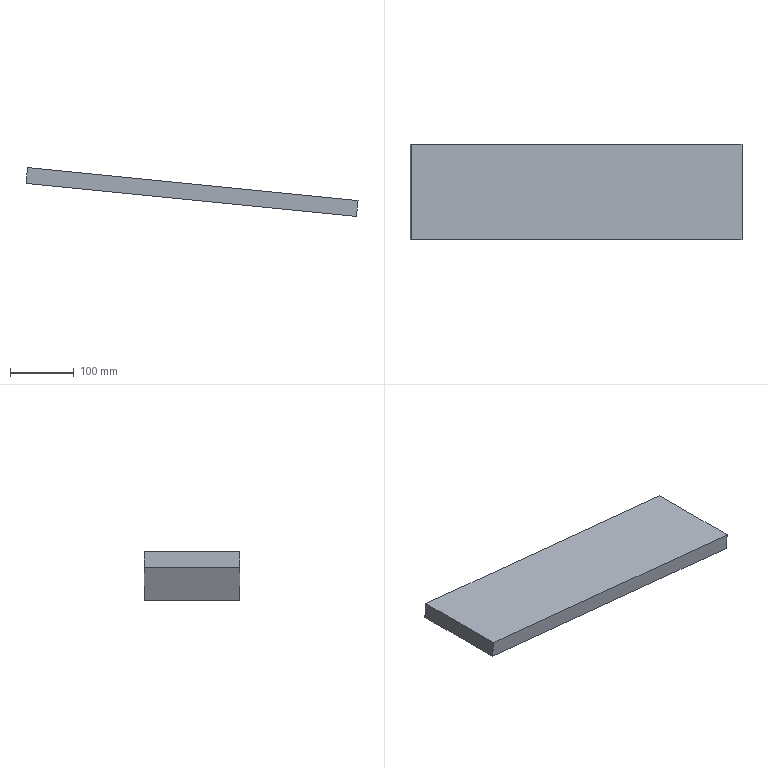Component | NX | MOVING_FRAME_BLOCK_1_2 | 1 solid | 6 faces | box 519.91 x 150 x 76.52 mm | volume 1950000 mm3 | plane 6
STEP:
#1=CARTESIAN_POINT('',(0.,0.,0.));
#2=DIRECTION('',(0.,0.,1.));
#3=DIRECTION('',(1.,0.,0.));
#4=AXIS2_PLACEMENT_3D('',#1,#2,#3);
#5=CARTESIAN_POINT('',(480.652,-7.5,574.818));
#6=VERTEX_POINT('',#5);
#7=CARTESIAN_POINT('',(478.169,-7.5,549.942));
#8=VERTEX_POINT('',#7);
#9=CARTESIAN_POINT('',(480.652,-7.5,574.818));
#10=DIRECTION('',(-0.09932,0.,-0.9951));
#11=VECTOR('',#10,1.);
#12=LINE('',#9,#11);
#13=CARTESIAN_POINT('',(998.081,-7.5,523.172));
#14=DIRECTION('',(0.,1.,0.));
#15=DIRECTION('',(0.09932,0.,0.9951));
#16=AXIS2_PLACEMENT_3D('',#13,#14,#15);
#17=PLANE('',#16);
#18=CARTESIAN_POINT('',(-0.,-520.));
#19=DIRECTION('',(-1.,0.));
#20=VECTOR('',#19,1.);
#21=LINE('',#18,#20);
#22=(GEOMETRIC_REPRESENTATION_CONTEXT(2)PARAMETRIC_REPRESENTATION_CONTEXT()REPRESENTATION_CONTEXT('',''));
#23=DEFINITIONAL_REPRESENTATION('',(#21),#22);
#24=PCURVE('',#17,#23);
#25=CARTESIAN_POINT('',(478.169,-7.5,549.942));
#26=DIRECTION('',(0.9951,0.,-0.09932));
#27=DIRECTION('',(-0.09932,0.,-0.9951));
#28=AXIS2_PLACEMENT_3D('',#25,#26,#27);
#29=PLANE('',#28);
#30=CARTESIAN_POINT('',(-25.,0.));
#31=DIRECTION('',(1.,0.));
#32=VECTOR('',#31,1.);
#33=LINE('',#30,#32);
#34=(GEOMETRIC_REPRESENTATION_CONTEXT(2)PARAMETRIC_REPRESENTATION_CONTEXT()REPRESENTATION_CONTEXT('',''));
#35=DEFINITIONAL_REPRESENTATION('',(#33),#34);
#36=PCURVE('',#29,#35);
#37=SURFACE_CURVE('',#12,(#24,#36),.PCURVE_S1.);
#38=EDGE_CURVE('',#6,#8,#37,.T.);
#39=ORIENTED_EDGE('',*,*,#38,.T.);
#40=CARTESIAN_POINT('',(995.598,-7.5,498.296));
#41=VERTEX_POINT('',#40);
#42=CARTESIAN_POINT('',(995.598,-7.5,498.296));
#43=DIRECTION('',(-0.9951,0.,0.09932));
#44=VECTOR('',#43,1.);
#45=LINE('',#42,#44);
#46=CARTESIAN_POINT('',(-25.,0.));
#47=DIRECTION('',(-0.,-1.));
#48=VECTOR('',#47,1.);
#49=LINE('',#46,#48);
#50=(GEOMETRIC_REPRESENTATION_CONTEXT(2)PARAMETRIC_REPRESENTATION_CONTEXT()REPRESENTATION_CONTEXT('',''));
#51=DEFINITIONAL_REPRESENTATION('',(#49),#50);
#52=PCURVE('',#17,#51);
#53=CARTESIAN_POINT('',(995.598,-7.5,498.296));
#54=DIRECTION('',(0.09932,0.,0.9951));
#55=DIRECTION('',(0.9951,0.,-0.09932));
#56=AXIS2_PLACEMENT_3D('',#53,#54,#55);
#57=PLANE('',#56);
#58=CARTESIAN_POINT('',(0.,0.));
#59=DIRECTION('',(-1.,0.));
#60=VECTOR('',#59,1.);
#61=LINE('',#58,#60);
#62=(GEOMETRIC_REPRESENTATION_CONTEXT(2)PARAMETRIC_REPRESENTATION_CONTEXT()REPRESENTATION_CONTEXT('',''));
#63=DEFINITIONAL_REPRESENTATION('',(#61),#62);
#64=PCURVE('',#57,#63);
#65=SURFACE_CURVE('',#45,(#52,#64),.PCURVE_S1.);
#66=EDGE_CURVE('',#41,#8,#65,.T.);
#67=ORIENTED_EDGE('',*,*,#66,.F.);
#68=CARTESIAN_POINT('',(998.081,-7.5,523.172));
#69=VERTEX_POINT('',#68);
#70=CARTESIAN_POINT('',(998.081,-7.5,523.172));
#71=DIRECTION('',(-0.09932,0.,-0.9951));
#72=VECTOR('',#71,1.);
#73=LINE('',#70,#72);
#74=CARTESIAN_POINT('',(0.,0.));
#75=DIRECTION('',(-1.,0.));
#76=VECTOR('',#75,1.);
#77=LINE('',#74,#76);
#78=(GEOMETRIC_REPRESENTATION_CONTEXT(2)PARAMETRIC_REPRESENTATION_CONTEXT()REPRESENTATION_CONTEXT('',''));
#79=DEFINITIONAL_REPRESENTATION('',(#77),#78);
#80=PCURVE('',#17,#79);
#81=CARTESIAN_POINT('',(995.598,-7.5,498.296));
#82=DIRECTION('',(0.9951,0.,-0.09932));
#83=DIRECTION('',(-0.09932,0.,-0.9951));
#84=AXIS2_PLACEMENT_3D('',#81,#82,#83);
#85=PLANE('',#84);
#86=CARTESIAN_POINT('',(-25.,0.));
#87=DIRECTION('',(1.,0.));
#88=VECTOR('',#87,1.);
#89=LINE('',#86,#88);
#90=(GEOMETRIC_REPRESENTATION_CONTEXT(2)PARAMETRIC_REPRESENTATION_CONTEXT()REPRESENTATION_CONTEXT('',''));
#91=DEFINITIONAL_REPRESENTATION('',(#89),#90);
#92=PCURVE('',#85,#91);
#93=SURFACE_CURVE('',#73,(#80,#92),.PCURVE_S1.);
#94=EDGE_CURVE('',#69,#41,#93,.T.);
#95=ORIENTED_EDGE('',*,*,#94,.F.);
#96=CARTESIAN_POINT('',(998.081,-7.5,523.172));
#97=DIRECTION('',(-0.9951,0.,0.09932));
#98=VECTOR('',#97,1.);
#99=LINE('',#96,#98);
#100=CARTESIAN_POINT('',(0.,0.));
#101=DIRECTION('',(-0.,-1.));
#102=VECTOR('',#101,1.);
#103=LINE('',#100,#102);
#104=(GEOMETRIC_REPRESENTATION_CONTEXT(2)PARAMETRIC_REPRESENTATION_CONTEXT()REPRESENTATION_CONTEXT('',''));
#105=DEFINITIONAL_REPRESENTATION('',(#103),#104);
#106=PCURVE('',#17,#105);
#107=CARTESIAN_POINT('',(998.081,142.5,523.172));
#108=DIRECTION('',(-0.09932,0.,-0.9951));
#109=DIRECTION('',(0.,1.,0.));
#110=AXIS2_PLACEMENT_3D('',#107,#108,#109);
#111=PLANE('',#110);
#112=CARTESIAN_POINT('',(-150.,-0.));
#113=DIRECTION('',(0.,-1.));
#114=VECTOR('',#113,1.);
#115=LINE('',#112,#114);
#116=(GEOMETRIC_REPRESENTATION_CONTEXT(2)PARAMETRIC_REPRESENTATION_CONTEXT()REPRESENTATION_CONTEXT('',''));
#117=DEFINITIONAL_REPRESENTATION('',(#115),#116);
#118=PCURVE('',#111,#117);
#119=SURFACE_CURVE('',#99,(#106,#118),.PCURVE_S1.);
#120=EDGE_CURVE('',#69,#6,#119,.T.);
#121=ORIENTED_EDGE('',*,*,#120,.T.);
#122=EDGE_LOOP('',(#39,#67,#95,#121));
#123=FACE_BOUND('',#122,.T.);
#124=ADVANCED_FACE('',(#123),#17,.F.);
#125=CARTESIAN_POINT('',(478.169,142.5,549.942));
#126=VERTEX_POINT('',#125);
#127=CARTESIAN_POINT('',(478.169,-7.5,549.942));
#128=DIRECTION('',(0.,1.,0.));
#129=VECTOR('',#128,1.);
#130=LINE('',#127,#129);
#131=CARTESIAN_POINT('',(-520.,0.));
#132=DIRECTION('',(0.,1.));
#133=VECTOR('',#132,1.);
#134=LINE('',#131,#133);
#135=(GEOMETRIC_REPRESENTATION_CONTEXT(2)PARAMETRIC_REPRESENTATION_CONTEXT()REPRESENTATION_CONTEXT('',''));
#136=DEFINITIONAL_REPRESENTATION('',(#134),#135);
#137=PCURVE('',#57,#136);
#138=CARTESIAN_POINT('',(0.,0.));
#139=DIRECTION('',(0.,1.));
#140=VECTOR('',#139,1.);
#141=LINE('',#138,#140);
#142=(GEOMETRIC_REPRESENTATION_CONTEXT(2)PARAMETRIC_REPRESENTATION_CONTEXT()REPRESENTATION_CONTEXT('',''));
#143=DEFINITIONAL_REPRESENTATION('',(#141),#142);
#144=PCURVE('',#29,#143);
#145=SURFACE_CURVE('',#130,(#137,#144),.PCURVE_S1.);
#146=EDGE_CURVE('',#8,#126,#145,.T.);
#147=ORIENTED_EDGE('',*,*,#146,.T.);
#148=CARTESIAN_POINT('',(995.598,142.5,498.296));
#149=VERTEX_POINT('',#148);
#150=CARTESIAN_POINT('',(995.598,142.5,498.296));
#151=DIRECTION('',(-0.9951,0.,0.09932));
#152=VECTOR('',#151,1.);
#153=LINE('',#150,#152);
#154=CARTESIAN_POINT('',(0.,150.));
#155=DIRECTION('',(-1.,0.));
#156=VECTOR('',#155,1.);
#157=LINE('',#154,#156);
#158=(GEOMETRIC_REPRESENTATION_CONTEXT(2)PARAMETRIC_REPRESENTATION_CONTEXT()REPRESENTATION_CONTEXT('',''));
#159=DEFINITIONAL_REPRESENTATION('',(#157),#158);
#160=PCURVE('',#57,#159);
#161=CARTESIAN_POINT('',(995.598,142.5,498.296));
#162=DIRECTION('',(0.,-1.,0.));
#163=DIRECTION('',(-0.09932,0.,-0.9951));
#164=AXIS2_PLACEMENT_3D('',#161,#162,#163);
#165=PLANE('',#164);
#166=CARTESIAN_POINT('',(0.,0.));
#167=DIRECTION('',(0.,-1.));
#168=VECTOR('',#167,1.);
#169=LINE('',#166,#168);
#170=(GEOMETRIC_REPRESENTATION_CONTEXT(2)PARAMETRIC_REPRESENTATION_CONTEXT()REPRESENTATION_CONTEXT('',''));
#171=DEFINITIONAL_REPRESENTATION('',(#169),#170);
#172=PCURVE('',#165,#171);
#173=SURFACE_CURVE('',#153,(#160,#172),.PCURVE_S1.);
#174=EDGE_CURVE('',#149,#126,#173,.T.);
#175=ORIENTED_EDGE('',*,*,#174,.F.);
#176=CARTESIAN_POINT('',(995.598,-7.5,498.296));
#177=DIRECTION('',(0.,1.,0.));
#178=VECTOR('',#177,1.);
#179=LINE('',#176,#178);
#180=CARTESIAN_POINT('',(0.,0.));
#181=DIRECTION('',(0.,1.));
#182=VECTOR('',#181,1.);
#183=LINE('',#180,#182);
#184=(GEOMETRIC_REPRESENTATION_CONTEXT(2)PARAMETRIC_REPRESENTATION_CONTEXT()REPRESENTATION_CONTEXT('',''));
#185=DEFINITIONAL_REPRESENTATION('',(#183),#184);
#186=PCURVE('',#57,#185);
#187=CARTESIAN_POINT('',(0.,0.));
#188=DIRECTION('',(0.,1.));
#189=VECTOR('',#188,1.);
#190=LINE('',#187,#189);
#191=(GEOMETRIC_REPRESENTATION_CONTEXT(2)PARAMETRIC_REPRESENTATION_CONTEXT()REPRESENTATION_CONTEXT('',''));
#192=DEFINITIONAL_REPRESENTATION('',(#190),#191);
#193=PCURVE('',#85,#192);
#194=SURFACE_CURVE('',#179,(#186,#193),.PCURVE_S1.);
#195=EDGE_CURVE('',#41,#149,#194,.T.);
#196=ORIENTED_EDGE('',*,*,#195,.F.);
#197=ORIENTED_EDGE('',*,*,#66,.T.);
#198=EDGE_LOOP('',(#147,#175,#196,#197));
#199=FACE_BOUND('',#198,.T.);
#200=ADVANCED_FACE('',(#199),#57,.F.);
#201=CARTESIAN_POINT('',(480.652,142.5,574.818));
#202=VERTEX_POINT('',#201);
#203=CARTESIAN_POINT('',(478.169,142.5,549.942));
#204=DIRECTION('',(0.09932,0.,0.9951));
#205=VECTOR('',#204,1.);
#206=LINE('',#203,#205);
#207=CARTESIAN_POINT('',(0.,-520.));
#208=DIRECTION('',(-1.,-0.));
#209=VECTOR('',#208,1.);
#210=LINE('',#207,#209);
#211=(GEOMETRIC_REPRESENTATION_CONTEXT(2)PARAMETRIC_REPRESENTATION_CONTEXT()REPRESENTATION_CONTEXT('',''));
#212=DEFINITIONAL_REPRESENTATION('',(#210),#211);
#213=PCURVE('',#165,#212);
#214=CARTESIAN_POINT('',(0.,150.));
#215=DIRECTION('',(-1.,0.));
#216=VECTOR('',#215,1.);
#217=LINE('',#214,#216);
#218=(GEOMETRIC_REPRESENTATION_CONTEXT(2)PARAMETRIC_REPRESENTATION_CONTEXT()REPRESENTATION_CONTEXT('',''));
#219=DEFINITIONAL_REPRESENTATION('',(#217),#218);
#220=PCURVE('',#29,#219);
#221=SURFACE_CURVE('',#206,(#213,#220),.PCURVE_S1.);
#222=EDGE_CURVE('',#126,#202,#221,.T.);
#223=ORIENTED_EDGE('',*,*,#222,.T.);
#224=CARTESIAN_POINT('',(998.081,142.5,523.172));
#225=VERTEX_POINT('',#224);
#226=CARTESIAN_POINT('',(998.081,142.5,523.172));
#227=DIRECTION('',(-0.9951,0.,0.09932));
#228=VECTOR('',#227,1.);
#229=LINE('',#226,#228);
#230=CARTESIAN_POINT('',(-25.,-0.));
#231=DIRECTION('',(0.,-1.));
#232=VECTOR('',#231,1.);
#233=LINE('',#230,#232);
#234=(GEOMETRIC_REPRESENTATION_CONTEXT(2)PARAMETRIC_REPRESENTATION_CONTEXT()REPRESENTATION_CONTEXT('',''));
#235=DEFINITIONAL_REPRESENTATION('',(#233),#234);
#236=PCURVE('',#165,#235);
#237=CARTESIAN_POINT('',(0.,0.));
#238=DIRECTION('',(0.,-1.));
#239=VECTOR('',#238,1.);
#240=LINE('',#237,#239);
#241=(GEOMETRIC_REPRESENTATION_CONTEXT(2)PARAMETRIC_REPRESENTATION_CONTEXT()REPRESENTATION_CONTEXT('',''));
#242=DEFINITIONAL_REPRESENTATION('',(#240),#241);
#243=PCURVE('',#111,#242);
#244=SURFACE_CURVE('',#229,(#236,#243),.PCURVE_S1.);
#245=EDGE_CURVE('',#225,#202,#244,.T.);
#246=ORIENTED_EDGE('',*,*,#245,.F.);
#247=CARTESIAN_POINT('',(995.598,142.5,498.296));
#248=DIRECTION('',(0.09932,0.,0.9951));
#249=VECTOR('',#248,1.);
#250=LINE('',#247,#249);
#251=CARTESIAN_POINT('',(0.,0.));
#252=DIRECTION('',(-1.,-0.));
#253=VECTOR('',#252,1.);
#254=LINE('',#251,#253);
#255=(GEOMETRIC_REPRESENTATION_CONTEXT(2)PARAMETRIC_REPRESENTATION_CONTEXT()REPRESENTATION_CONTEXT('',''));
#256=DEFINITIONAL_REPRESENTATION('',(#254),#255);
#257=PCURVE('',#165,#256);
#258=CARTESIAN_POINT('',(0.,150.));
#259=DIRECTION('',(-1.,0.));
#260=VECTOR('',#259,1.);
#261=LINE('',#258,#260);
#262=(GEOMETRIC_REPRESENTATION_CONTEXT(2)PARAMETRIC_REPRESENTATION_CONTEXT()REPRESENTATION_CONTEXT('',''));
#263=DEFINITIONAL_REPRESENTATION('',(#261),#262);
#264=PCURVE('',#85,#263);
#265=SURFACE_CURVE('',#250,(#257,#264),.PCURVE_S1.);
#266=EDGE_CURVE('',#149,#225,#265,.T.);
#267=ORIENTED_EDGE('',*,*,#266,.F.);
#268=ORIENTED_EDGE('',*,*,#174,.T.);
#269=EDGE_LOOP('',(#223,#246,#267,#268));
#270=FACE_BOUND('',#269,.T.);
#271=ADVANCED_FACE('',(#270),#165,.F.);
#272=CARTESIAN_POINT('',(480.652,142.5,574.818));
#273=DIRECTION('',(-0.,-1.,-0.));
#274=VECTOR('',#273,1.);
#275=LINE('',#272,#274);
#276=CARTESIAN_POINT('',(0.,-520.));
#277=DIRECTION('',(-1.,-0.));
#278=VECTOR('',#277,1.);
#279=LINE('',#276,#278);
#280=(GEOMETRIC_REPRESENTATION_CONTEXT(2)PARAMETRIC_REPRESENTATION_CONTEXT()REPRESENTATION_CONTEXT('',''));
#281=DEFINITIONAL_REPRESENTATION('',(#279),#280);
#282=PCURVE('',#111,#281);
#283=CARTESIAN_POINT('',(-25.,150.));
#284=DIRECTION('',(0.,-1.));
#285=VECTOR('',#284,1.);
#286=LINE('',#283,#285);
#287=(GEOMETRIC_REPRESENTATION_CONTEXT(2)PARAMETRIC_REPRESENTATION_CONTEXT()REPRESENTATION_CONTEXT('',''));
#288=DEFINITIONAL_REPRESENTATION('',(#286),#287);
#289=PCURVE('',#29,#288);
#290=SURFACE_CURVE('',#275,(#282,#289),.PCURVE_S1.);
#291=EDGE_CURVE('',#202,#6,#290,.T.);
#292=ORIENTED_EDGE('',*,*,#291,.T.);
#293=ORIENTED_EDGE('',*,*,#120,.F.);
#294=CARTESIAN_POINT('',(998.081,142.5,523.172));
#295=DIRECTION('',(-0.,-1.,-0.));
#296=VECTOR('',#295,1.);
#297=LINE('',#294,#296);
#298=CARTESIAN_POINT('',(0.,0.));
#299=DIRECTION('',(-1.,-0.));
#300=VECTOR('',#299,1.);
#301=LINE('',#298,#300);
#302=(GEOMETRIC_REPRESENTATION_CONTEXT(2)PARAMETRIC_REPRESENTATION_CONTEXT()REPRESENTATION_CONTEXT('',''));
#303=DEFINITIONAL_REPRESENTATION('',(#301),#302);
#304=PCURVE('',#111,#303);
#305=CARTESIAN_POINT('',(-25.,150.));
#306=DIRECTION('',(0.,-1.));
#307=VECTOR('',#306,1.);
#308=LINE('',#305,#307);
#309=(GEOMETRIC_REPRESENTATION_CONTEXT(2)PARAMETRIC_REPRESENTATION_CONTEXT()REPRESENTATION_CONTEXT('',''));
#310=DEFINITIONAL_REPRESENTATION('',(#308),#309);
#311=PCURVE('',#85,#310);
#312=SURFACE_CURVE('',#297,(#304,#311),.PCURVE_S1.);
#313=EDGE_CURVE('',#225,#69,#312,.T.);
#314=ORIENTED_EDGE('',*,*,#313,.F.);
#315=ORIENTED_EDGE('',*,*,#245,.T.);
#316=EDGE_LOOP('',(#292,#293,#314,#315));
#317=FACE_BOUND('',#316,.T.);
#318=ADVANCED_FACE('',(#317),#111,.F.);
#319=ORIENTED_EDGE('',*,*,#94,.T.);
#320=ORIENTED_EDGE('',*,*,#195,.T.);
#321=ORIENTED_EDGE('',*,*,#266,.T.);
#322=ORIENTED_EDGE('',*,*,#313,.T.);
#323=EDGE_LOOP('',(#319,#320,#321,#322));
#324=FACE_BOUND('',#323,.T.);
#325=ADVANCED_FACE('',(#324),#85,.T.);
#326=ORIENTED_EDGE('',*,*,#38,.F.);
#327=ORIENTED_EDGE('',*,*,#291,.F.);
#328=ORIENTED_EDGE('',*,*,#222,.F.);
#329=ORIENTED_EDGE('',*,*,#146,.F.);
#330=EDGE_LOOP('',(#326,#327,#328,#329));
#331=FACE_BOUND('',#330,.T.);
#332=ADVANCED_FACE('',(#331),#29,.F.);
#333=CLOSED_SHELL('',(#124,#200,#271,#318,#325,#332));
#334=MANIFOLD_SOLID_BREP('',#333);
#335=(LENGTH_UNIT()NAMED_UNIT(*)SI_UNIT(.MILLI.,.METRE.));
#336=UNCERTAINTY_MEASURE_WITH_UNIT(LENGTH_MEASURE(0.0000001),#335,'','');
#337=(NAMED_UNIT(*)PLANE_ANGLE_UNIT()SI_UNIT($,.RADIAN.));
#338=(NAMED_UNIT(*)SI_UNIT($,.STERADIAN.)SOLID_ANGLE_UNIT());
#339=(GEOMETRIC_REPRESENTATION_CONTEXT(3)GLOBAL_UNCERTAINTY_ASSIGNED_CONTEXT((#336))GLOBAL_UNIT_ASSIGNED_CONTEXT((#335,#337,#338))REPRESENTATION_CONTEXT('',''));
#340=ADVANCED_BREP_SHAPE_REPRESENTATION('',(#4,#334),#339);